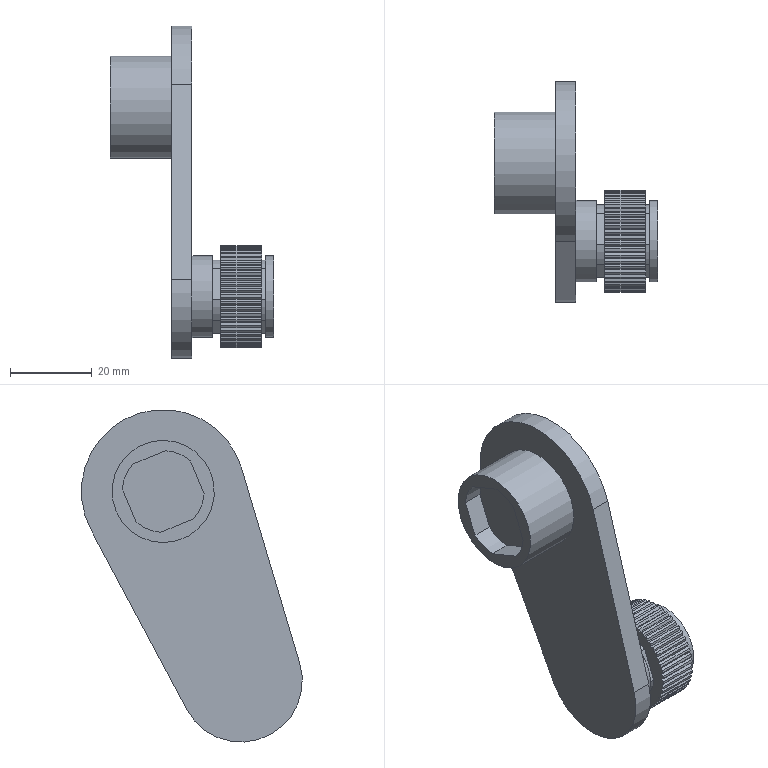Component | NX | SHE_JI-7 | 2 solids | 190 faces | volume 27194 mm3 | plane 123 | cylinder 67 | commonest cylinder face diameters 25 x51 20 x6 18 x5 18.4 x3 30 x1 40 x1